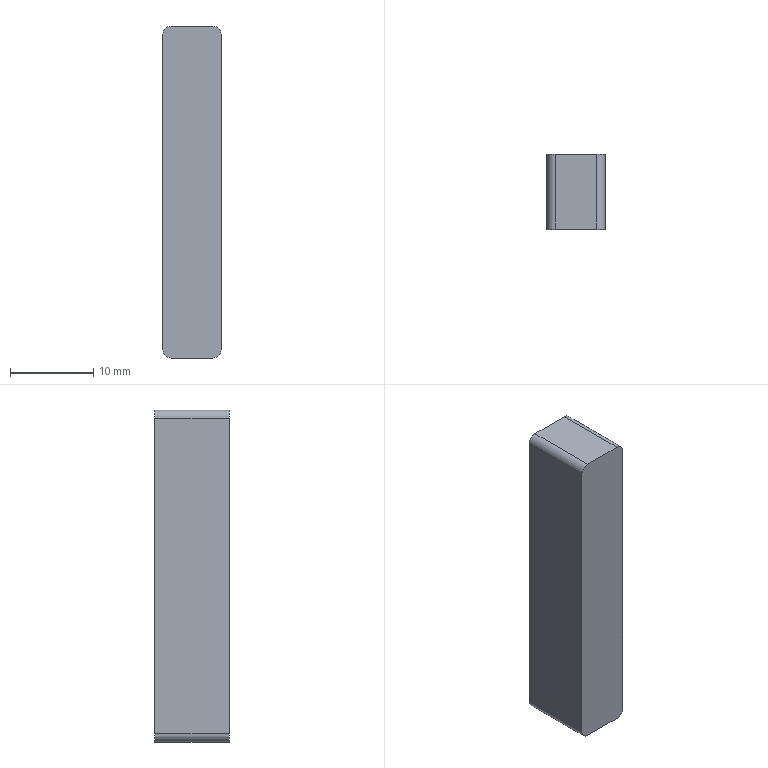CAM job | Mastercam | mm | 7 operations | part box 7 x 9 x 40
1. Facing | 20 - 63 平铣刀
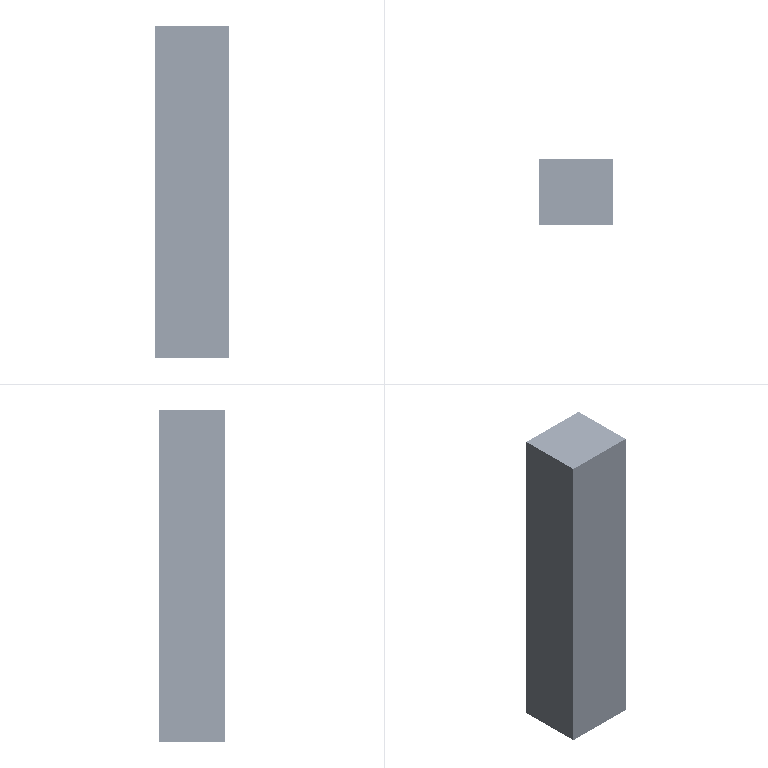2. Contour (Ramp) | 12 - 12 平铣刀
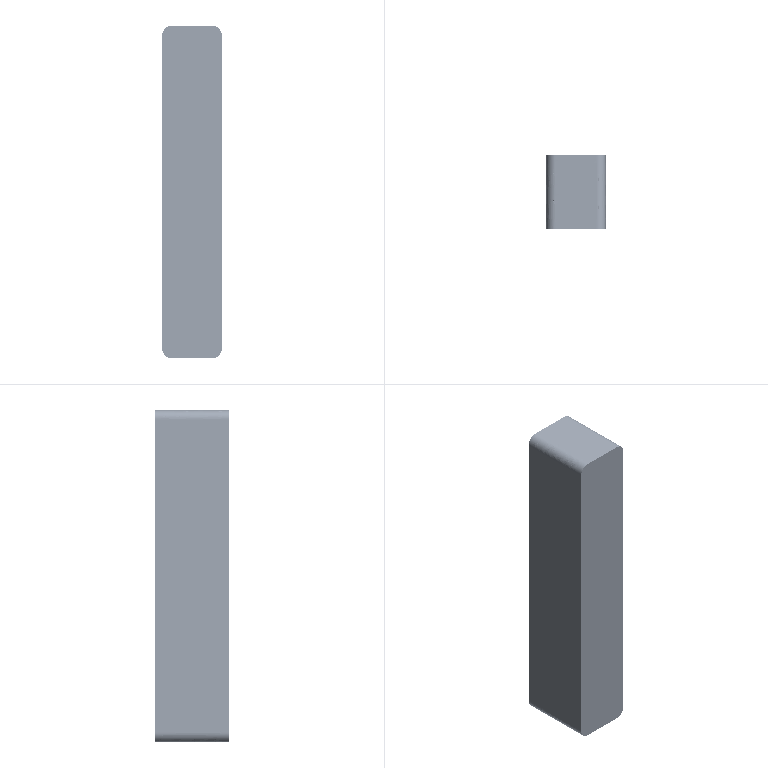3. Contour (2D) | 12 - 12 平铣刀
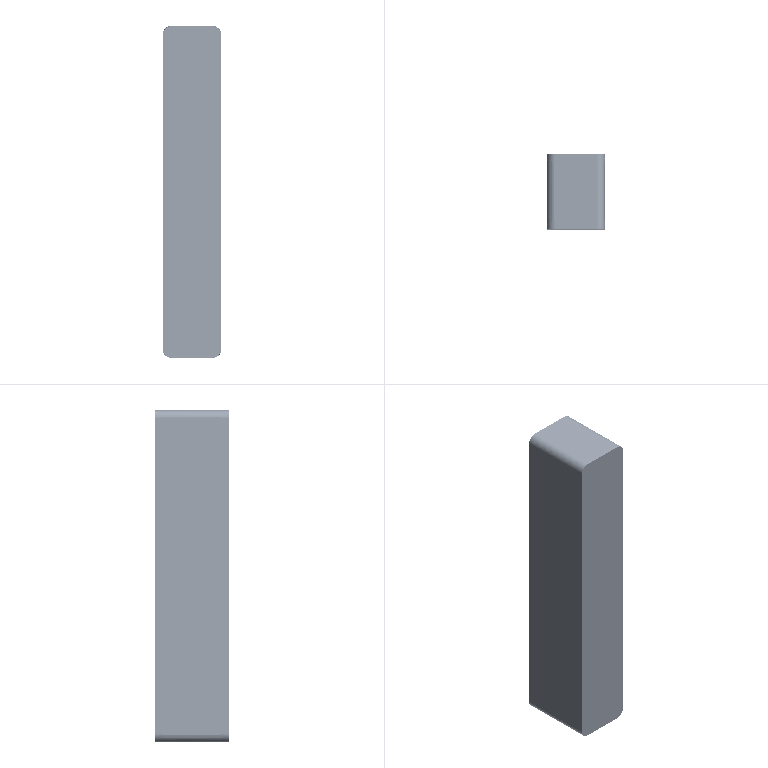4. Drill/Counterbore | 7 - 4 倒角刀
5. Contour (2D chamfer) | 7 - 4 倒角刀
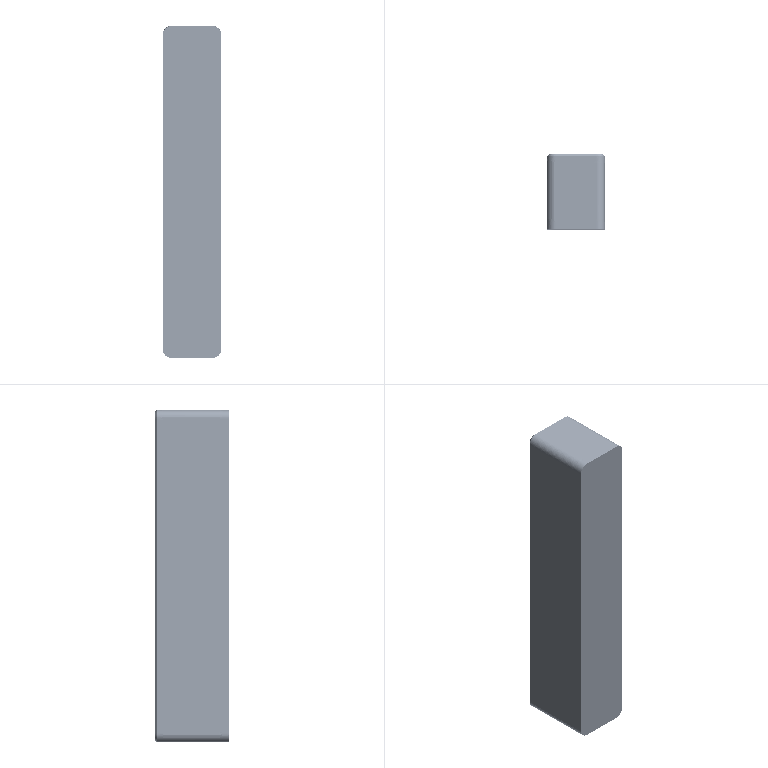6. Facing | 20 - 63 平铣刀
7. Contour (2D chamfer) | 7 - 4 倒角刀